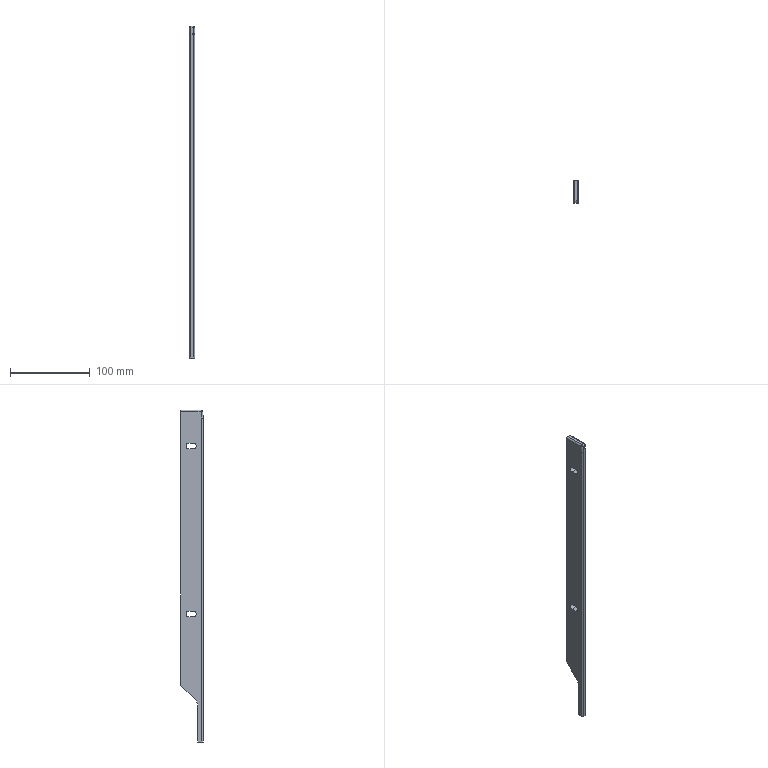Component | SolidWorks | WirePressingUnitPressingPlate-1 | 1 solid | 30 faces | box 7 x 28 x 415 mm | volume 70543 mm3 | plane 13 | cylinder 13 | sphere 4 | commonest cylinder face diameters 4 x8 7 x4 20 x1
STEP:
#1=COLOUR_RGB('',0.7922,0.8196,0.9333);
#2=FILL_AREA_STYLE_COLOUR('',#1);
#3=FILL_AREA_STYLE('',(#2));
#4=SURFACE_STYLE_FILL_AREA(#3);
#5=SURFACE_SIDE_STYLE('',(#4));
#6=SURFACE_STYLE_USAGE(.BOTH.,#5);
#7=PRESENTATION_STYLE_ASSIGNMENT((#6));
#8=CARTESIAN_POINT('',(-0.3085,-0.6154,-14.209));
#9=VERTEX_POINT('',#8);
#10=CARTESIAN_POINT('',(-0.3085,-0.8123,-14.209));
#11=VERTEX_POINT('',#10);
#12=CARTESIAN_POINT('',(-0.3085,0.2113,-14.209));
#13=DIRECTION('',(0.,-1.,-0.));
#14=VECTOR('',#13,39.37);
#15=LINE('',#12,#14);
#16=EDGE_CURVE('',#9,#11,#15,.T.);
#17=ORIENTED_EDGE('',*,*,#16,.F.);
#18=CARTESIAN_POINT('',(-0.03288,-0.6154,-14.209));
#19=VERTEX_POINT('',#18);
#20=CARTESIAN_POINT('',(-0.03288,-0.6154,-14.209));
#21=DIRECTION('',(-1.,-0.,-0.));
#22=VECTOR('',#21,39.37);
#23=LINE('',#20,#22);
#24=EDGE_CURVE('',#19,#9,#23,.T.);
#25=ORIENTED_EDGE('',*,*,#24,.F.);
#26=CARTESIAN_POINT('',(-0.03288,-0.8123,-14.209));
#27=VERTEX_POINT('',#26);
#28=CARTESIAN_POINT('',(-0.03288,0.2113,-14.209));
#29=DIRECTION('',(0.,-1.,-0.));
#30=VECTOR('',#29,39.37);
#31=LINE('',#28,#30);
#32=EDGE_CURVE('',#19,#27,#31,.T.);
#33=ORIENTED_EDGE('',*,*,#32,.T.);
#34=CARTESIAN_POINT('',(-0.1116,-0.891,-14.209));
#35=VERTEX_POINT('',#34);
#36=CARTESIAN_POINT('',(-0.1116,-0.8123,-14.209));
#37=DIRECTION('',(0.,0.,-1.));
#38=DIRECTION('',(1.,0.,0.));
#39=AXIS2_PLACEMENT_3D('',#36,#37,#38);
#40=CIRCLE('',#39,0.07874);
#41=EDGE_CURVE('',#27,#35,#40,.T.);
#42=ORIENTED_EDGE('',*,*,#41,.T.);
#43=CARTESIAN_POINT('',(-0.2297,-0.891,-14.209));
#44=VERTEX_POINT('',#43);
#45=CARTESIAN_POINT('',(-0.3085,-0.891,-14.209));
#46=DIRECTION('',(1.,0.,0.));
#47=VECTOR('',#46,39.37);
#48=LINE('',#45,#47);
#49=EDGE_CURVE('',#44,#35,#48,.T.);
#50=ORIENTED_EDGE('',*,*,#49,.F.);
#51=CARTESIAN_POINT('',(-0.2297,-0.8123,-14.209));
#52=DIRECTION('',(0.,0.,-1.));
#53=DIRECTION('',(1.,0.,0.));
#54=AXIS2_PLACEMENT_3D('',#51,#52,#53);
#55=CIRCLE('',#54,0.07874);
#56=EDGE_CURVE('',#44,#11,#55,.T.);
#57=ORIENTED_EDGE('',*,*,#56,.T.);
#58=EDGE_LOOP('',(#17,#25,#33,#42,#50,#57));
#59=FACE_OUTER_BOUND('',#58,.T.);
#60=CARTESIAN_POINT('',(-0.3085,0.2113,-14.209));
#61=DIRECTION('',(-0.,-0.,1.));
#62=DIRECTION('',(1.,0.,0.));
#63=AXIS2_PLACEMENT_3D('',#60,#61,#62);
#64=PLANE('',#63);
#65=ADVANCED_FACE('',(#59),#64,.F.);
#66=ORIENTED_EDGE('',*,*,#49,.T.);
#67=CARTESIAN_POINT('',(-0.1116,-0.891,1.732));
#68=VERTEX_POINT('',#67);
#69=CARTESIAN_POINT('',(-0.1116,-0.891,-14.209));
#70=DIRECTION('',(-0.,-0.,1.));
#71=VECTOR('',#70,39.37);
#72=LINE('',#69,#71);
#73=EDGE_CURVE('',#35,#68,#72,.T.);
#74=ORIENTED_EDGE('',*,*,#73,.T.);
#75=CARTESIAN_POINT('',(-0.2297,-0.891,1.732));
#76=VERTEX_POINT('',#75);
#77=CARTESIAN_POINT('',(-0.3085,-0.891,1.732));
#78=DIRECTION('',(-1.,-0.,-0.));
#79=VECTOR('',#78,39.37);
#80=LINE('',#77,#79);
#81=EDGE_CURVE('',#68,#76,#80,.T.);
#82=ORIENTED_EDGE('',*,*,#81,.T.);
#83=CARTESIAN_POINT('',(-0.2297,-0.891,-14.209));
#84=DIRECTION('',(0.,0.,-1.));
#85=VECTOR('',#84,39.37);
#86=LINE('',#83,#85);
#87=EDGE_CURVE('',#76,#44,#86,.T.);
#88=ORIENTED_EDGE('',*,*,#87,.T.);
#89=EDGE_LOOP('',(#66,#74,#82,#88));
#90=FACE_OUTER_BOUND('',#89,.T.);
#91=CARTESIAN_POINT('',(-0.3085,-0.891,-14.209));
#92=DIRECTION('',(-0.,1.,0.));
#93=DIRECTION('',(-1.,-0.,-0.));
#94=AXIS2_PLACEMENT_3D('',#91,#92,#93);
#95=PLANE('',#94);
#96=ADVANCED_FACE('',(#90),#95,.F.);
#97=CARTESIAN_POINT('',(-0.2297,-0.8907,1.739));
#98=VERTEX_POINT('',#97);
#99=CARTESIAN_POINT('',(-0.1116,-0.8907,1.739));
#100=VERTEX_POINT('',#99);
#101=CARTESIAN_POINT('',(-0.3085,-0.8907,1.739));
#102=DIRECTION('',(1.,0.,0.));
#103=VECTOR('',#102,39.37);
#104=LINE('',#101,#103);
#105=EDGE_CURVE('',#98,#100,#104,.T.);
#106=ORIENTED_EDGE('',*,*,#105,.T.);
#107=CARTESIAN_POINT('',(-0.1116,-0.8629,2.057));
#108=VERTEX_POINT('',#107);
#109=CARTESIAN_POINT('',(-0.1116,-0.8566,2.129));
#110=DIRECTION('',(-0.,0.08716,0.9962));
#111=VECTOR('',#110,39.37);
#112=LINE('',#109,#111);
#113=EDGE_CURVE('',#100,#108,#112,.T.);
#114=ORIENTED_EDGE('',*,*,#113,.T.);
#115=CARTESIAN_POINT('',(-0.2297,-0.8629,2.057));
#116=VERTEX_POINT('',#115);
#117=CARTESIAN_POINT('',(-0.3085,-0.8629,2.057));
#118=DIRECTION('',(-1.,-0.,-0.));
#119=VECTOR('',#118,39.37);
#120=LINE('',#117,#119);
#121=EDGE_CURVE('',#108,#116,#120,.T.);
#122=ORIENTED_EDGE('',*,*,#121,.T.);
#123=CARTESIAN_POINT('',(-0.2297,-0.8907,1.739));
#124=DIRECTION('',(0.,-0.08716,-0.9962));
#125=VECTOR('',#124,39.37);
#126=LINE('',#123,#125);
#127=EDGE_CURVE('',#116,#98,#126,.T.);
#128=ORIENTED_EDGE('',*,*,#127,.T.);
#129=EDGE_LOOP('',(#106,#114,#122,#128));
#130=FACE_OUTER_BOUND('',#129,.T.);
#131=CARTESIAN_POINT('',(-0.3085,-0.8566,2.129));
#132=DIRECTION('',(-0.,0.9962,-0.08716));
#133=DIRECTION('',(0.,-0.08716,-0.9962));
#134=AXIS2_PLACEMENT_3D('',#131,#132,#133);
#135=PLANE('',#134);
#136=ADVANCED_FACE('',(#130),#135,.F.);
#137=CARTESIAN_POINT('',(-0.2297,-0.7844,2.129));
#138=VERTEX_POINT('',#137);
#139=CARTESIAN_POINT('',(-0.1116,-0.7844,2.129));
#140=VERTEX_POINT('',#139);
#141=CARTESIAN_POINT('',(-0.3085,-0.7844,2.129));
#142=DIRECTION('',(1.,0.,0.));
#143=VECTOR('',#142,39.37);
#144=LINE('',#141,#143);
#145=EDGE_CURVE('',#138,#140,#144,.T.);
#146=ORIENTED_EDGE('',*,*,#145,.T.);
#147=CARTESIAN_POINT('',(-0.1116,0.2113,2.129));
#148=VERTEX_POINT('',#147);
#149=CARTESIAN_POINT('',(-0.1116,0.2113,2.129));
#150=DIRECTION('',(-0.,1.,0.));
#151=VECTOR('',#150,39.37);
#152=LINE('',#149,#151);
#153=EDGE_CURVE('',#140,#148,#152,.T.);
#154=ORIENTED_EDGE('',*,*,#153,.T.);
#155=CARTESIAN_POINT('',(-0.2297,0.2113,2.129));
#156=VERTEX_POINT('',#155);
#157=CARTESIAN_POINT('',(-0.3085,0.2113,2.129));
#158=DIRECTION('',(1.,0.,0.));
#159=VECTOR('',#158,39.37);
#160=LINE('',#157,#159);
#161=EDGE_CURVE('',#156,#148,#160,.T.);
#162=ORIENTED_EDGE('',*,*,#161,.F.);
#163=CARTESIAN_POINT('',(-0.2297,-0.7844,2.129));
#164=DIRECTION('',(0.,-1.,-0.));
#165=VECTOR('',#164,39.37);
#166=LINE('',#163,#165);
#167=EDGE_CURVE('',#156,#138,#166,.T.);
#168=ORIENTED_EDGE('',*,*,#167,.T.);
#169=EDGE_LOOP('',(#146,#154,#162,#168));
#170=FACE_OUTER_BOUND('',#169,.T.);
#171=CARTESIAN_POINT('',(-0.3085,0.2113,2.129));
#172=DIRECTION('',(0.,0.,-1.));
#173=DIRECTION('',(-1.,-0.,-0.));
#174=AXIS2_PLACEMENT_3D('',#171,#172,#173);
#175=PLANE('',#174);
#176=ADVANCED_FACE('',(#170),#175,.F.);
#177=CARTESIAN_POINT('',(-0.03288,0.2113,2.051));
#178=VERTEX_POINT('',#177);
#179=CARTESIAN_POINT('',(-0.03288,0.2113,-11.414));
#180=VERTEX_POINT('',#179);
#181=CARTESIAN_POINT('',(-0.03288,0.2113,-14.209));
#182=DIRECTION('',(0.,0.,-1.));
#183=VECTOR('',#182,39.37);
#184=LINE('',#181,#183);
#185=EDGE_CURVE('',#178,#180,#184,.T.);
#186=ORIENTED_EDGE('',*,*,#185,.T.);
#187=CARTESIAN_POINT('',(-0.3085,0.2113,-11.414));
#188=VERTEX_POINT('',#187);
#189=CARTESIAN_POINT('',(-0.03288,0.2113,-11.414));
#190=DIRECTION('',(-1.,-0.,-0.));
#191=VECTOR('',#190,39.37);
#192=LINE('',#189,#191);
#193=EDGE_CURVE('',#180,#188,#192,.T.);
#194=ORIENTED_EDGE('',*,*,#193,.T.);
#195=CARTESIAN_POINT('',(-0.3085,0.2113,2.051));
#196=VERTEX_POINT('',#195);
#197=CARTESIAN_POINT('',(-0.3085,0.2113,-14.209));
#198=DIRECTION('',(0.,0.,-1.));
#199=VECTOR('',#198,39.37);
#200=LINE('',#197,#199);
#201=EDGE_CURVE('',#196,#188,#200,.T.);
#202=ORIENTED_EDGE('',*,*,#201,.F.);
#203=CARTESIAN_POINT('',(-0.2297,0.2113,2.051));
#204=DIRECTION('',(-0.,1.,0.));
#205=DIRECTION('',(1.,0.,0.));
#206=AXIS2_PLACEMENT_3D('',#203,#204,#205);
#207=CIRCLE('',#206,0.07874);
#208=EDGE_CURVE('',#196,#156,#207,.T.);
#209=ORIENTED_EDGE('',*,*,#208,.T.);
#210=ORIENTED_EDGE('',*,*,#161,.T.);
#211=CARTESIAN_POINT('',(-0.1116,0.2113,2.051));
#212=DIRECTION('',(-0.,1.,0.));
#213=DIRECTION('',(1.,0.,0.));
#214=AXIS2_PLACEMENT_3D('',#211,#212,#213);
#215=CIRCLE('',#214,0.07874);
#216=EDGE_CURVE('',#148,#178,#215,.T.);
#217=ORIENTED_EDGE('',*,*,#216,.T.);
#218=EDGE_LOOP('',(#186,#194,#202,#209,#210,#217));
#219=FACE_OUTER_BOUND('',#218,.T.);
#220=CARTESIAN_POINT('',(-0.3085,0.2113,-14.209));
#221=DIRECTION('',(0.,-1.,-0.));
#222=DIRECTION('',(1.,0.,0.));
#223=AXIS2_PLACEMENT_3D('',#220,#221,#222);
#224=PLANE('',#223);
#225=ADVANCED_FACE('',(#219),#224,.F.);
#226=CARTESIAN_POINT('',(-0.3085,-0.5001,-12.125));
#227=VERTEX_POINT('',#226);
#228=CARTESIAN_POINT('',(-0.3085,0.2113,-11.414));
#229=DIRECTION('',(-0.,0.7071,0.7071));
#230=VECTOR('',#229,39.37);
#231=LINE('',#228,#230);
#232=EDGE_CURVE('',#227,#188,#231,.T.);
#233=ORIENTED_EDGE('',*,*,#232,.F.);
#234=CARTESIAN_POINT('',(-0.3085,-0.6154,-12.404));
#235=VERTEX_POINT('',#234);
#236=CARTESIAN_POINT('',(-0.3085,-0.2217,-12.404));
#237=DIRECTION('',(-1.,-0.,-0.));
#238=DIRECTION('',(0.,0.,1.));
#239=AXIS2_PLACEMENT_3D('',#236,#237,#238);
#240=CIRCLE('',#239,0.3937);
#241=EDGE_CURVE('',#235,#227,#240,.T.);
#242=ORIENTED_EDGE('',*,*,#241,.F.);
#243=CARTESIAN_POINT('',(-0.3085,-0.6154,-14.209));
#244=DIRECTION('',(-0.,-0.,1.));
#245=VECTOR('',#244,39.37);
#246=LINE('',#243,#245);
#247=EDGE_CURVE('',#9,#235,#246,.T.);
#248=ORIENTED_EDGE('',*,*,#247,.F.);
#249=ORIENTED_EDGE('',*,*,#16,.T.);
#250=CARTESIAN_POINT('',(-0.3085,-0.8123,1.732));
#251=VERTEX_POINT('',#250);
#252=CARTESIAN_POINT('',(-0.3085,-0.8123,1.732));
#253=DIRECTION('',(-0.,-0.,1.));
#254=VECTOR('',#253,39.37);
#255=LINE('',#252,#254);
#256=EDGE_CURVE('',#11,#251,#255,.T.);
#257=ORIENTED_EDGE('',*,*,#256,.T.);
#258=CARTESIAN_POINT('',(-0.3085,-0.7844,2.051));
#259=VERTEX_POINT('',#258);
#260=CARTESIAN_POINT('',(-0.3085,-0.7844,2.051));
#261=DIRECTION('',(-0.,0.08716,0.9962));
#262=VECTOR('',#261,39.37);
#263=LINE('',#260,#262);
#264=EDGE_CURVE('',#251,#259,#263,.T.);
#265=ORIENTED_EDGE('',*,*,#264,.T.);
#266=CARTESIAN_POINT('',(-0.3085,0.2113,2.051));
#267=DIRECTION('',(-0.,1.,0.));
#268=VECTOR('',#267,39.37);
#269=LINE('',#266,#268);
#270=EDGE_CURVE('',#259,#196,#269,.T.);
#271=ORIENTED_EDGE('',*,*,#270,.T.);
#272=ORIENTED_EDGE('',*,*,#201,.T.);
#273=EDGE_LOOP('',(#233,#242,#248,#249,#257,#265,#271,#272));
#274=FACE_OUTER_BOUND('',#273,.T.);
#275=CARTESIAN_POINT('',(-0.3085,-0.1824,-7.772));
#276=VERTEX_POINT('',#275);
#277=CARTESIAN_POINT('',(-0.3085,-0.1824,-8.048));
#278=VERTEX_POINT('',#277);
#279=CARTESIAN_POINT('',(-0.3085,-0.1824,-7.91));
#280=DIRECTION('',(-1.,-0.,-0.));
#281=DIRECTION('',(0.,0.,1.));
#282=AXIS2_PLACEMENT_3D('',#279,#280,#281);
#283=CIRCLE('',#282,0.1378);
#284=EDGE_CURVE('',#276,#278,#283,.T.);
#285=ORIENTED_EDGE('',*,*,#284,.F.);
#286=CARTESIAN_POINT('',(-0.3085,-0.4186,-7.772));
#287=VERTEX_POINT('',#286);
#288=CARTESIAN_POINT('',(-0.3085,-0.1824,-7.772));
#289=DIRECTION('',(-0.,1.,0.));
#290=VECTOR('',#289,39.37);
#291=LINE('',#288,#290);
#292=EDGE_CURVE('',#287,#276,#291,.T.);
#293=ORIENTED_EDGE('',*,*,#292,.F.);
#294=CARTESIAN_POINT('',(-0.3085,-0.4186,-8.048));
#295=VERTEX_POINT('',#294);
#296=CARTESIAN_POINT('',(-0.3085,-0.4186,-7.91));
#297=DIRECTION('',(-1.,-0.,-0.));
#298=DIRECTION('',(0.,0.,1.));
#299=AXIS2_PLACEMENT_3D('',#296,#297,#298);
#300=CIRCLE('',#299,0.1378);
#301=EDGE_CURVE('',#295,#287,#300,.T.);
#302=ORIENTED_EDGE('',*,*,#301,.F.);
#303=CARTESIAN_POINT('',(-0.3085,-0.1824,-8.048));
#304=DIRECTION('',(0.,-1.,-0.));
#305=VECTOR('',#304,39.37);
#306=LINE('',#303,#305);
#307=EDGE_CURVE('',#278,#295,#306,.T.);
#308=ORIENTED_EDGE('',*,*,#307,.F.);
#309=EDGE_LOOP('',(#285,#293,#302,#308));
#310=FACE_BOUND('',#309,.T.);
#311=CARTESIAN_POINT('',(-0.3085,-0.1824,0.4955));
#312=VERTEX_POINT('',#311);
#313=CARTESIAN_POINT('',(-0.3085,-0.1824,0.2199));
#314=VERTEX_POINT('',#313);
#315=CARTESIAN_POINT('',(-0.3085,-0.1824,0.3577));
#316=DIRECTION('',(-1.,-0.,-0.));
#317=DIRECTION('',(0.,0.,1.));
#318=AXIS2_PLACEMENT_3D('',#315,#316,#317);
#319=CIRCLE('',#318,0.1378);
#320=EDGE_CURVE('',#312,#314,#319,.T.);
#321=ORIENTED_EDGE('',*,*,#320,.F.);
#322=CARTESIAN_POINT('',(-0.3085,-0.4186,0.4955));
#323=VERTEX_POINT('',#322);
#324=CARTESIAN_POINT('',(-0.3085,-0.1824,0.4955));
#325=DIRECTION('',(-0.,1.,0.));
#326=VECTOR('',#325,39.37);
#327=LINE('',#324,#326);
#328=EDGE_CURVE('',#323,#312,#327,.T.);
#329=ORIENTED_EDGE('',*,*,#328,.F.);
#330=CARTESIAN_POINT('',(-0.3085,-0.4186,0.2199));
#331=VERTEX_POINT('',#330);
#332=CARTESIAN_POINT('',(-0.3085,-0.4186,0.3577));
#333=DIRECTION('',(-1.,-0.,-0.));
#334=DIRECTION('',(0.,0.,1.));
#335=AXIS2_PLACEMENT_3D('',#332,#333,#334);
#336=CIRCLE('',#335,0.1378);
#337=EDGE_CURVE('',#331,#323,#336,.T.);
#338=ORIENTED_EDGE('',*,*,#337,.F.);
#339=CARTESIAN_POINT('',(-0.3085,-0.1824,0.2199));
#340=DIRECTION('',(0.,-1.,-0.));
#341=VECTOR('',#340,39.37);
#342=LINE('',#339,#341);
#343=EDGE_CURVE('',#314,#331,#342,.T.);
#344=ORIENTED_EDGE('',*,*,#343,.F.);
#345=EDGE_LOOP('',(#321,#329,#338,#344));
#346=FACE_BOUND('',#345,.T.);
#347=CARTESIAN_POINT('',(-0.3085,-0.3398,-6.04));
#348=DIRECTION('',(-1.,-0.,-0.));
#349=DIRECTION('',(-0.,-0.,1.));
#350=AXIS2_PLACEMENT_3D('',#347,#348,#349);
#351=PLANE('',#350);
#352=ADVANCED_FACE('',(#274,#310,#346),#351,.T.);
#353=CARTESIAN_POINT('',(-0.03288,-0.4186,-7.772));
#354=VERTEX_POINT('',#353);
#355=CARTESIAN_POINT('',(-0.03288,-0.1824,-7.772));
#356=VERTEX_POINT('',#355);
#357=CARTESIAN_POINT('',(-0.03288,-0.3398,-7.772));
#358=DIRECTION('',(-0.,1.,0.));
#359=VECTOR('',#358,39.37);
#360=LINE('',#357,#359);
#361=EDGE_CURVE('',#354,#356,#360,.T.);
#362=ORIENTED_EDGE('',*,*,#361,.T.);
#363=CARTESIAN_POINT('',(-0.03288,-0.1824,-8.048));
#364=VERTEX_POINT('',#363);
#365=CARTESIAN_POINT('',(-0.03288,-0.1824,-7.91));
#366=DIRECTION('',(-1.,-0.,-0.));
#367=DIRECTION('',(0.,0.,1.));
#368=AXIS2_PLACEMENT_3D('',#365,#366,#367);
#369=CIRCLE('',#368,0.1378);
#370=EDGE_CURVE('',#356,#364,#369,.T.);
#371=ORIENTED_EDGE('',*,*,#370,.T.);
#372=CARTESIAN_POINT('',(-0.03288,-0.4186,-8.048));
#373=VERTEX_POINT('',#372);
#374=CARTESIAN_POINT('',(-0.03288,-0.3398,-8.048));
#375=DIRECTION('',(0.,-1.,-0.));
#376=VECTOR('',#375,39.37);
#377=LINE('',#374,#376);
#378=EDGE_CURVE('',#364,#373,#377,.T.);
#379=ORIENTED_EDGE('',*,*,#378,.T.);
#380=CARTESIAN_POINT('',(-0.03288,-0.4186,-7.91));
#381=DIRECTION('',(-1.,-0.,-0.));
#382=DIRECTION('',(0.,0.,1.));
#383=AXIS2_PLACEMENT_3D('',#380,#381,#382);
#384=CIRCLE('',#383,0.1378);
#385=EDGE_CURVE('',#373,#354,#384,.T.);
#386=ORIENTED_EDGE('',*,*,#385,.T.);
#387=EDGE_LOOP('',(#362,#371,#379,#386));
#388=FACE_BOUND('',#387,.T.);
#389=CARTESIAN_POINT('',(-0.03288,-0.4186,0.4955));
#390=VERTEX_POINT('',#389);
#391=CARTESIAN_POINT('',(-0.03288,-0.1824,0.4955));
#392=VERTEX_POINT('',#391);
#393=CARTESIAN_POINT('',(-0.03288,-0.3398,0.4955));
#394=DIRECTION('',(-0.,1.,0.));
#395=VECTOR('',#394,39.37);
#396=LINE('',#393,#395);
#397=EDGE_CURVE('',#390,#392,#396,.T.);
#398=ORIENTED_EDGE('',*,*,#397,.T.);
#399=CARTESIAN_POINT('',(-0.03288,-0.1824,0.2199));
#400=VERTEX_POINT('',#399);
#401=CARTESIAN_POINT('',(-0.03288,-0.1824,0.3577));
#402=DIRECTION('',(-1.,-0.,-0.));
#403=DIRECTION('',(0.,0.,1.));
#404=AXIS2_PLACEMENT_3D('',#401,#402,#403);
#405=CIRCLE('',#404,0.1378);
#406=EDGE_CURVE('',#392,#400,#405,.T.);
#407=ORIENTED_EDGE('',*,*,#406,.T.);
#408=CARTESIAN_POINT('',(-0.03288,-0.4186,0.2199));
#409=VERTEX_POINT('',#408);
#410=CARTESIAN_POINT('',(-0.03288,-0.3398,0.2199));
#411=DIRECTION('',(0.,-1.,-0.));
#412=VECTOR('',#411,39.37);
#413=LINE('',#410,#412);
#414=EDGE_CURVE('',#400,#409,#413,.T.);
#415=ORIENTED_EDGE('',*,*,#414,.T.);
#416=CARTESIAN_POINT('',(-0.03288,-0.4186,0.3577));
#417=DIRECTION('',(-1.,-0.,-0.));
#418=DIRECTION('',(0.,0.,1.));
#419=AXIS2_PLACEMENT_3D('',#416,#417,#418);
#420=CIRCLE('',#419,0.1378);
#421=EDGE_CURVE('',#409,#390,#420,.T.);
#422=ORIENTED_EDGE('',*,*,#421,.T.);
#423=EDGE_LOOP('',(#398,#407,#415,#422));
#424=FACE_BOUND('',#423,.T.);
#425=CARTESIAN_POINT('',(-0.03288,-0.6154,-12.404));
#426=VERTEX_POINT('',#425);
#427=CARTESIAN_POINT('',(-0.03288,-0.5001,-12.125));
#428=VERTEX_POINT('',#427);
#429=CARTESIAN_POINT('',(-0.03288,-0.2217,-12.404));
#430=DIRECTION('',(-1.,-0.,-0.));
#431=DIRECTION('',(-0.,0.,1.));
#432=AXIS2_PLACEMENT_3D('',#429,#430,#431);
#433=CIRCLE('',#432,0.3937);
#434=EDGE_CURVE('',#426,#428,#433,.T.);
#435=ORIENTED_EDGE('',*,*,#434,.T.);
#436=CARTESIAN_POINT('',(-0.03288,0.2113,-11.414));
#437=DIRECTION('',(-0.,0.7071,0.7071));
#438=VECTOR('',#437,39.37);
#439=LINE('',#436,#438);
#440=EDGE_CURVE('',#428,#180,#439,.T.);
#441=ORIENTED_EDGE('',*,*,#440,.T.);
#442=ORIENTED_EDGE('',*,*,#185,.F.);
#443=CARTESIAN_POINT('',(-0.03288,-0.7844,2.051));
#444=VERTEX_POINT('',#443);
#445=CARTESIAN_POINT('',(-0.03288,-0.3398,2.051));
#446=DIRECTION('',(0.,-1.,-0.));
#447=VECTOR('',#446,39.37);
#448=LINE('',#445,#447);
#449=EDGE_CURVE('',#178,#444,#448,.T.);
#450=ORIENTED_EDGE('',*,*,#449,.T.);
#451=CARTESIAN_POINT('',(-0.03288,-0.8123,1.732));
#452=VERTEX_POINT('',#451);
#453=CARTESIAN_POINT('',(-0.03288,-1.483,-5.94));
#454=DIRECTION('',(0.,-0.08716,-0.9962));
#455=VECTOR('',#454,39.37);
#456=LINE('',#453,#455);
#457=EDGE_CURVE('',#444,#452,#456,.T.);
#458=ORIENTED_EDGE('',*,*,#457,.T.);
#459=CARTESIAN_POINT('',(-0.03288,-0.8123,-6.04));
#460=DIRECTION('',(0.,0.,-1.));
#461=VECTOR('',#460,39.37);
#462=LINE('',#459,#461);
#463=EDGE_CURVE('',#452,#27,#462,.T.);
#464=ORIENTED_EDGE('',*,*,#463,.T.);
#465=ORIENTED_EDGE('',*,*,#32,.F.);
#466=CARTESIAN_POINT('',(-0.03288,-0.6154,-14.209));
#467=DIRECTION('',(-0.,-0.,1.));
#468=VECTOR('',#467,39.37);
#469=LINE('',#466,#468);
#470=EDGE_CURVE('',#19,#426,#469,.T.);
#471=ORIENTED_EDGE('',*,*,#470,.T.);
#472=EDGE_LOOP('',(#435,#441,#442,#450,#458,#464,#465,#471));
#473=FACE_OUTER_BOUND('',#472,.T.);
#474=CARTESIAN_POINT('',(-0.03288,-0.3398,-6.04));
#475=DIRECTION('',(-1.,-0.,-0.));
#476=DIRECTION('',(-0.,-0.,1.));
#477=AXIS2_PLACEMENT_3D('',#474,#475,#476);
#478=PLANE('',#477);
#479=ADVANCED_FACE('',(#388,#424,#473),#478,.F.);
#480=ORIENTED_EDGE('',*,*,#81,.F.);
#481=CARTESIAN_POINT('',(-0.1116,-0.8123,1.732));
#482=DIRECTION('',(-1.,-0.,-0.));
#483=DIRECTION('',(0.,0.,-1.));
#484=AXIS2_PLACEMENT_3D('',#481,#482,#483);
#485=CIRCLE('',#484,0.07874);
#486=EDGE_CURVE('',#68,#100,#485,.T.);
#487=ORIENTED_EDGE('',*,*,#486,.T.);
#488=ORIENTED_EDGE('',*,*,#105,.F.);
#489=CARTESIAN_POINT('',(-0.2297,-0.8123,1.732));
#490=DIRECTION('',(1.,0.,0.));
#491=DIRECTION('',(0.,0.,-1.));
#492=AXIS2_PLACEMENT_3D('',#489,#490,#491);
#493=CIRCLE('',#492,0.07874);
#494=EDGE_CURVE('',#98,#76,#493,.T.);
#495=ORIENTED_EDGE('',*,*,#494,.T.);
#496=EDGE_LOOP('',(#480,#487,#488,#495));
#497=FACE_OUTER_BOUND('',#496,.T.);
#498=CARTESIAN_POINT('',(-0.3085,-0.8123,1.732));
#499=DIRECTION('',(1.,0.,0.));
#500=DIRECTION('',(0.,0.,-1.));
#501=AXIS2_PLACEMENT_3D('',#498,#499,#500);
#502=CYLINDRICAL_SURFACE('',#501,0.07874);
#503=ADVANCED_FACE('',(#497),#502,.T.);
#504=ORIENTED_EDGE('',*,*,#121,.F.);
#505=CARTESIAN_POINT('',(-0.1116,-0.7844,2.051));
#506=DIRECTION('',(-1.,-0.,-0.));
#507=DIRECTION('',(0.,0.,-1.));
#508=AXIS2_PLACEMENT_3D('',#505,#506,#507);
#509=CIRCLE('',#508,0.07874);
#510=EDGE_CURVE('',#108,#140,#509,.T.);
#511=ORIENTED_EDGE('',*,*,#510,.T.);
#512=ORIENTED_EDGE('',*,*,#145,.F.);
#513=CARTESIAN_POINT('',(-0.2297,-0.7844,2.051));
#514=DIRECTION('',(1.,0.,0.));
#515=DIRECTION('',(0.,0.,-1.));
#516=AXIS2_PLACEMENT_3D('',#513,#514,#515);
#517=CIRCLE('',#516,0.07874);
#518=EDGE_CURVE('',#138,#116,#517,.T.);
#519=ORIENTED_EDGE('',*,*,#518,.T.);
#520=EDGE_LOOP('',(#504,#511,#512,#519));
#521=FACE_OUTER_BOUND('',#520,.T.);
#522=CARTESIAN_POINT('',(-0.3085,-0.7844,2.051));
#523=DIRECTION('',(1.,0.,0.));
#524=DIRECTION('',(0.,0.,-1.));
#525=AXIS2_PLACEMENT_3D('',#522,#523,#524);
#526=CYLINDRICAL_SURFACE('',#525,0.07874);
#527=ADVANCED_FACE('',(#521),#526,.T.);
#528=CARTESIAN_POINT('',(-0.1116,-0.8123,1.732));
#529=DIRECTION('',(-0.,-0.,1.));
#530=DIRECTION('',(1.,0.,0.));
#531=AXIS2_PLACEMENT_3D('',#528,#529,#530);
#532=CIRCLE('',#531,0.07874);
#533=EDGE_CURVE('',#68,#452,#532,.T.);
#534=ORIENTED_EDGE('',*,*,#533,.F.);
#535=ORIENTED_EDGE('',*,*,#73,.F.);
#536=ORIENTED_EDGE('',*,*,#41,.F.);
#537=ORIENTED_EDGE('',*,*,#463,.F.);
#538=EDGE_LOOP('',(#534,#535,#536,#537));
#539=FACE_OUTER_BOUND('',#538,.T.);
#540=CARTESIAN_POINT('',(-0.1116,-0.8123,-14.209));
#541=DIRECTION('',(-0.,-0.,1.));
#542=DIRECTION('',(1.,0.,0.));
#543=AXIS2_PLACEMENT_3D('',#540,#541,#542);
#544=CYLINDRICAL_SURFACE('',#543,0.07874);
#545=ADVANCED_FACE('',(#539),#544,.T.);
#546=ORIENTED_EDGE('',*,*,#486,.F.);
#547=ORIENTED_EDGE('',*,*,#533,.T.);
#548=CARTESIAN_POINT('',(-0.1116,-0.8123,1.732));
#549=DIRECTION('',(-0.,0.08716,0.9962));
#550=DIRECTION('',(0.,0.9962,-0.08716));
#551=AXIS2_PLACEMENT_3D('',#548,#549,#550);
#552=CIRCLE('',#551,0.07874);
#553=EDGE_CURVE('',#100,#452,#552,.T.);
#554=ORIENTED_EDGE('',*,*,#553,.F.);
#555=EDGE_LOOP('',(#546,#547,#554));
#556=FACE_OUTER_BOUND('',#555,.T.);
#557=CARTESIAN_POINT('',(-0.1116,-0.8123,1.732));
#558=DIRECTION('',(-0.,1.,0.));
#559=DIRECTION('',(0.,0.,1.));
#560=AXIS2_PLACEMENT_3D('',#557,#558,#559);
#561=SPHERICAL_SURFACE('',#560,0.07874);
#562=ADVANCED_FACE('',(#556),#561,.T.);
#563=CARTESIAN_POINT('',(-0.1116,-0.7844,2.051));
#564=DIRECTION('',(0.,0.08716,0.9962));
#565=DIRECTION('',(0.,0.9962,-0.08716));
#566=AXIS2_PLACEMENT_3D('',#563,#564,#565);
#567=CIRCLE('',#566,0.07874);
#568=EDGE_CURVE('',#108,#444,#567,.T.);
#569=ORIENTED_EDGE('',*,*,#568,.F.);
#570=ORIENTED_EDGE('',*,*,#113,.F.);
#571=ORIENTED_EDGE('',*,*,#553,.T.);
#572=ORIENTED_EDGE('',*,*,#457,.F.);
#573=EDGE_LOOP('',(#569,#570,#571,#572));
#574=FACE_OUTER_BOUND('',#573,.T.);
#575=CARTESIAN_POINT('',(-0.1116,-0.7781,2.122));
#576=DIRECTION('',(-0.,0.08716,0.9962));
#577=DIRECTION('',(0.,0.9962,-0.08716));
#578=AXIS2_PLACEMENT_3D('',#575,#576,#577);
#579=CYLINDRICAL_SURFACE('',#578,0.07874);
#580=ADVANCED_FACE('',(#574),#579,.T.);
#581=ORIENTED_EDGE('',*,*,#510,.F.);
#582=ORIENTED_EDGE('',*,*,#568,.T.);
#583=CARTESIAN_POINT('',(-0.1116,-0.7844,2.051));
#584=DIRECTION('',(-0.,1.,0.));
#585=DIRECTION('',(-1.,0.,0.));
#586=AXIS2_PLACEMENT_3D('',#583,#584,#585);
#587=CIRCLE('',#586,0.07874);
#588=EDGE_CURVE('',#140,#444,#587,.T.);
#589=ORIENTED_EDGE('',*,*,#588,.F.);
#590=EDGE_LOOP('',(#581,#582,#589));
#591=FACE_OUTER_BOUND('',#590,.T.);
#592=CARTESIAN_POINT('',(-0.1116,-0.7844,2.051));
#593=DIRECTION('',(-0.,1.,0.));
#594=DIRECTION('',(0.,0.,1.));
#595=AXIS2_PLACEMENT_3D('',#592,#593,#594);
#596=SPHERICAL_SURFACE('',#595,0.07874);
#597=ADVANCED_FACE('',(#591),#596,.T.);
#598=ORIENTED_EDGE('',*,*,#588,.T.);
#599=ORIENTED_EDGE('',*,*,#449,.F.);
#600=ORIENTED_EDGE('',*,*,#216,.F.);
#601=ORIENTED_EDGE('',*,*,#153,.F.);
#602=EDGE_LOOP('',(#598,#599,#600,#601));
#603=FACE_OUTER_BOUND('',#602,.T.);
#604=CARTESIAN_POINT('',(-0.1116,0.2113,2.051));
#605=DIRECTION('',(-0.,1.,0.));
#606=DIRECTION('',(-1.,0.,0.));
#607=AXIS2_PLACEMENT_3D('',#604,#605,#606);
#608=CYLINDRICAL_SURFACE('',#607,0.07874);
#609=ADVANCED_FACE('',(#603),#608,.T.);
#610=ORIENTED_EDGE('',*,*,#56,.F.);
#611=ORIENTED_EDGE('',*,*,#87,.F.);
#612=CARTESIAN_POINT('',(-0.2297,-0.8123,1.732));
#613=DIRECTION('',(-0.,-0.,1.));
#614=DIRECTION('',(1.,0.,0.));
#615=AXIS2_PLACEMENT_3D('',#612,#613,#614);
#616=CIRCLE('',#615,0.07874);
#617=EDGE_CURVE('',#251,#76,#616,.T.);
#618=ORIENTED_EDGE('',*,*,#617,.F.);
#619=ORIENTED_EDGE('',*,*,#256,.F.);
#620=EDGE_LOOP('',(#610,#611,#618,#619));
#621=FACE_OUTER_BOUND('',#620,.T.);
#622=CARTESIAN_POINT('',(-0.2297,-0.8123,-6.04));
#623=DIRECTION('',(0.,0.,-1.));
#624=DIRECTION('',(-1.,0.,0.));
#625=AXIS2_PLACEMENT_3D('',#622,#623,#624);
#626=CYLINDRICAL_SURFACE('',#625,0.07874);
#627=ADVANCED_FACE('',(#621),#626,.T.);
#628=ORIENTED_EDGE('',*,*,#617,.T.);
#629=ORIENTED_EDGE('',*,*,#494,.F.);
#630=CARTESIAN_POINT('',(-0.2297,-0.8123,1.732));
#631=DIRECTION('',(-0.,0.08716,0.9962));
#632=DIRECTION('',(0.,0.9962,-0.08716));
#633=AXIS2_PLACEMENT_3D('',#630,#631,#632);
#634=CIRCLE('',#633,0.07874);
#635=EDGE_CURVE('',#251,#98,#634,.T.);
#636=ORIENTED_EDGE('',*,*,#635,.F.);
#637=EDGE_LOOP('',(#628,#629,#636));
#638=FACE_OUTER_BOUND('',#637,.T.);
#639=CARTESIAN_POINT('',(-0.2297,-0.8123,1.732));
#640=DIRECTION('',(-0.,1.,0.));
#641=DIRECTION('',(0.,0.,1.));
#642=AXIS2_PLACEMENT_3D('',#639,#640,#641);
#643=SPHERICAL_SURFACE('',#642,0.07874);
#644=ADVANCED_FACE('',(#638),#643,.T.);
#645=ORIENTED_EDGE('',*,*,#635,.T.);
#646=ORIENTED_EDGE('',*,*,#127,.F.);
#647=CARTESIAN_POINT('',(-0.2297,-0.7844,2.051));
#648=DIRECTION('',(-0.,0.08716,0.9962));
#649=DIRECTION('',(0.,0.9962,-0.08716));
#650=AXIS2_PLACEMENT_3D('',#647,#648,#649);
#651=CIRCLE('',#650,0.07874);
#652=EDGE_CURVE('',#259,#116,#651,.T.);
#653=ORIENTED_EDGE('',*,*,#652,.F.);
#654=ORIENTED_EDGE('',*,*,#264,.F.);
#655=EDGE_LOOP('',(#645,#646,#653,#654));
#656=FACE_OUTER_BOUND('',#655,.T.);
#657=CARTESIAN_POINT('',(-0.2297,-1.483,-5.94));
#658=DIRECTION('',(0.,-0.08716,-0.9962));
#659=DIRECTION('',(0.,-0.9962,0.08716));
#660=AXIS2_PLACEMENT_3D('',#657,#658,#659);
#661=CYLINDRICAL_SURFACE('',#660,0.07874);
#662=ADVANCED_FACE('',(#656),#661,.T.);
#663=ORIENTED_EDGE('',*,*,#652,.T.);
#664=ORIENTED_EDGE('',*,*,#518,.F.);
#665=CARTESIAN_POINT('',(-0.2297,-0.7844,2.051));
#666=DIRECTION('',(-0.,1.,0.));
#667=DIRECTION('',(-1.,0.,0.));
#668=AXIS2_PLACEMENT_3D('',#665,#666,#667);
#669=CIRCLE('',#668,0.07874);
#670=EDGE_CURVE('',#259,#138,#669,.T.);
#671=ORIENTED_EDGE('',*,*,#670,.F.);
#672=EDGE_LOOP('',(#663,#664,#671));
#673=FACE_OUTER_BOUND('',#672,.T.);
#674=CARTESIAN_POINT('',(-0.2297,-0.7844,2.051));
#675=DIRECTION('',(-0.,1.,0.));
#676=DIRECTION('',(0.,0.,1.));
#677=AXIS2_PLACEMENT_3D('',#674,#675,#676);
#678=SPHERICAL_SURFACE('',#677,0.07874);
#679=ADVANCED_FACE('',(#673),#678,.T.);
#680=ORIENTED_EDGE('',*,*,#670,.T.);
#681=ORIENTED_EDGE('',*,*,#167,.F.);
#682=ORIENTED_EDGE('',*,*,#208,.F.);
#683=ORIENTED_EDGE('',*,*,#270,.F.);
#684=EDGE_LOOP('',(#680,#681,#682,#683));
#685=FACE_OUTER_BOUND('',#684,.T.);
#686=CARTESIAN_POINT('',(-0.2297,-0.3398,2.051));
#687=DIRECTION('',(0.,-1.,-0.));
#688=DIRECTION('',(1.,0.,0.));
#689=AXIS2_PLACEMENT_3D('',#686,#687,#688);
#690=CYLINDRICAL_SURFACE('',#689,0.07874);
#691=ADVANCED_FACE('',(#685),#690,.T.);
#692=CARTESIAN_POINT('',(0.08523,-0.1824,0.4955));
#693=DIRECTION('',(-1.,-0.,-0.));
#694=VECTOR('',#693,39.37);
#695=LINE('',#692,#694);
#696=EDGE_CURVE('',#392,#312,#695,.T.);
#697=ORIENTED_EDGE('',*,*,#696,.T.);
#698=ORIENTED_EDGE('',*,*,#320,.T.);
#699=CARTESIAN_POINT('',(0.08523,-0.1824,0.2199));
#700=DIRECTION('',(-1.,-0.,-0.));
#701=VECTOR('',#700,39.37);
#702=LINE('',#699,#701);
#703=EDGE_CURVE('',#400,#314,#702,.T.);
#704=ORIENTED_EDGE('',*,*,#703,.F.);
#705=ORIENTED_EDGE('',*,*,#406,.F.);
#706=EDGE_LOOP('',(#697,#698,#704,#705));
#707=FACE_OUTER_BOUND('',#706,.T.);
#708=CARTESIAN_POINT('',(0.08523,-0.1824,0.3577));
#709=DIRECTION('',(-1.,-0.,-0.));
#710=DIRECTION('',(0.,0.,1.));
#711=AXIS2_PLACEMENT_3D('',#708,#709,#710);
#712=CYLINDRICAL_SURFACE('',#711,0.1378);
#713=ADVANCED_FACE('',(#707),#712,.F.);
#714=CARTESIAN_POINT('',(0.08523,-0.4186,0.4955));
#715=DIRECTION('',(-1.,-0.,-0.));
#716=VECTOR('',#715,39.37);
#717=LINE('',#714,#716);
#718=EDGE_CURVE('',#390,#323,#717,.T.);
#719=ORIENTED_EDGE('',*,*,#718,.T.);
#720=ORIENTED_EDGE('',*,*,#328,.T.);
#721=ORIENTED_EDGE('',*,*,#696,.F.);
#722=ORIENTED_EDGE('',*,*,#397,.F.);
#723=EDGE_LOOP('',(#719,#720,#721,#722));
#724=FACE_OUTER_BOUND('',#723,.T.);
#725=CARTESIAN_POINT('',(0.08523,-0.1824,0.4955));
#726=DIRECTION('',(-0.,-0.,1.));
#727=DIRECTION('',(1.,0.,0.));
#728=AXIS2_PLACEMENT_3D('',#725,#726,#727);
#729=PLANE('',#728);
#730=ADVANCED_FACE('',(#724),#729,.F.);
#731=CARTESIAN_POINT('',(0.08523,-0.4186,0.2199));
#732=DIRECTION('',(-1.,-0.,-0.));
#733=VECTOR('',#732,39.37);
#734=LINE('',#731,#733);
#735=EDGE_CURVE('',#409,#331,#734,.T.);
#736=ORIENTED_EDGE('',*,*,#735,.T.);
#737=ORIENTED_EDGE('',*,*,#337,.T.);
#738=ORIENTED_EDGE('',*,*,#718,.F.);
#739=ORIENTED_EDGE('',*,*,#421,.F.);
#740=EDGE_LOOP('',(#736,#737,#738,#739));
#741=FACE_OUTER_BOUND('',#740,.T.);
#742=CARTESIAN_POINT('',(0.08523,-0.4186,0.3577));
#743=DIRECTION('',(-1.,-0.,-0.));
#744=DIRECTION('',(0.,0.,1.));
#745=AXIS2_PLACEMENT_3D('',#742,#743,#744);
#746=CYLINDRICAL_SURFACE('',#745,0.1378);
#747=ADVANCED_FACE('',(#741),#746,.F.);
#748=ORIENTED_EDGE('',*,*,#703,.T.);
#749=ORIENTED_EDGE('',*,*,#343,.T.);
#750=ORIENTED_EDGE('',*,*,#735,.F.);
#751=ORIENTED_EDGE('',*,*,#414,.F.);
#752=EDGE_LOOP('',(#748,#749,#750,#751));
#753=FACE_OUTER_BOUND('',#752,.T.);
#754=CARTESIAN_POINT('',(0.08523,-0.1824,0.2199));
#755=DIRECTION('',(0.,0.,-1.));
#756=DIRECTION('',(-1.,-0.,-0.));
#757=AXIS2_PLACEMENT_3D('',#754,#755,#756);
#758=PLANE('',#757);
#759=ADVANCED_FACE('',(#753),#758,.F.);
#760=CARTESIAN_POINT('',(0.08523,-0.1824,-7.772));
#761=DIRECTION('',(-1.,-0.,-0.));
#762=VECTOR('',#761,39.37);
#763=LINE('',#760,#762);
#764=EDGE_CURVE('',#356,#276,#763,.T.);
#765=ORIENTED_EDGE('',*,*,#764,.T.);
#766=ORIENTED_EDGE('',*,*,#284,.T.);
#767=CARTESIAN_POINT('',(0.08523,-0.1824,-8.048));
#768=DIRECTION('',(-1.,-0.,-0.));
#769=VECTOR('',#768,39.37);
#770=LINE('',#767,#769);
#771=EDGE_CURVE('',#364,#278,#770,.T.);
#772=ORIENTED_EDGE('',*,*,#771,.F.);
#773=ORIENTED_EDGE('',*,*,#370,.F.);
#774=EDGE_LOOP('',(#765,#766,#772,#773));
#775=FACE_OUTER_BOUND('',#774,.T.);
#776=CARTESIAN_POINT('',(0.08523,-0.1824,-7.91));
#777=DIRECTION('',(-1.,-0.,-0.));
#778=DIRECTION('',(0.,0.,1.));
#779=AXIS2_PLACEMENT_3D('',#776,#777,#778);
#780=CYLINDRICAL_SURFACE('',#779,0.1378);
#781=ADVANCED_FACE('',(#775),#780,.F.);
#782=CARTESIAN_POINT('',(0.08523,-0.4186,-7.772));
#783=DIRECTION('',(-1.,-0.,-0.));
#784=VECTOR('',#783,39.37);
#785=LINE('',#782,#784);
#786=EDGE_CURVE('',#354,#287,#785,.T.);
#787=ORIENTED_EDGE('',*,*,#786,.T.);
#788=ORIENTED_EDGE('',*,*,#292,.T.);
#789=ORIENTED_EDGE('',*,*,#764,.F.);
#790=ORIENTED_EDGE('',*,*,#361,.F.);
#791=EDGE_LOOP('',(#787,#788,#789,#790));
#792=FACE_OUTER_BOUND('',#791,.T.);
#793=CARTESIAN_POINT('',(0.08523,-0.1824,-7.772));
#794=DIRECTION('',(-0.,-0.,1.));
#795=DIRECTION('',(1.,0.,0.));
#796=AXIS2_PLACEMENT_3D('',#793,#794,#795);
#797=PLANE('',#796);
#798=ADVANCED_FACE('',(#792),#797,.F.);
#799=CARTESIAN_POINT('',(0.08523,-0.4186,-8.048));
#800=DIRECTION('',(-1.,-0.,-0.));
#801=VECTOR('',#800,39.37);
#802=LINE('',#799,#801);
#803=EDGE_CURVE('',#373,#295,#802,.T.);
#804=ORIENTED_EDGE('',*,*,#803,.T.);
#805=ORIENTED_EDGE('',*,*,#301,.T.);
#806=ORIENTED_EDGE('',*,*,#786,.F.);
#807=ORIENTED_EDGE('',*,*,#385,.F.);
#808=EDGE_LOOP('',(#804,#805,#806,#807));
#809=FACE_OUTER_BOUND('',#808,.T.);
#810=CARTESIAN_POINT('',(0.08523,-0.4186,-7.91));
#811=DIRECTION('',(-1.,-0.,-0.));
#812=DIRECTION('',(0.,0.,1.));
#813=AXIS2_PLACEMENT_3D('',#810,#811,#812);
#814=CYLINDRICAL_SURFACE('',#813,0.1378);
#815=ADVANCED_FACE('',(#809),#814,.F.);
#816=ORIENTED_EDGE('',*,*,#771,.T.);
#817=ORIENTED_EDGE('',*,*,#307,.T.);
#818=ORIENTED_EDGE('',*,*,#803,.F.);
#819=ORIENTED_EDGE('',*,*,#378,.F.);
#820=EDGE_LOOP('',(#816,#817,#818,#819));
#821=FACE_OUTER_BOUND('',#820,.T.);
#822=CARTESIAN_POINT('',(0.08523,-0.1824,-8.048));
#823=DIRECTION('',(0.,0.,-1.));
#824=DIRECTION('',(-1.,-0.,-0.));
#825=AXIS2_PLACEMENT_3D('',#822,#823,#824);
#826=PLANE('',#825);
#827=ADVANCED_FACE('',(#821),#826,.F.);
#828=ORIENTED_EDGE('',*,*,#232,.T.);
#829=ORIENTED_EDGE('',*,*,#193,.F.);
#830=ORIENTED_EDGE('',*,*,#440,.F.);
#831=CARTESIAN_POINT('',(-0.03288,-0.5001,-12.125));
#832=DIRECTION('',(-1.,-0.,-0.));
#833=VECTOR('',#832,39.37);
#834=LINE('',#831,#833);
#835=EDGE_CURVE('',#428,#227,#834,.T.);
#836=ORIENTED_EDGE('',*,*,#835,.T.);
#837=EDGE_LOOP('',(#828,#829,#830,#836));
#838=FACE_OUTER_BOUND('',#837,.T.);
#839=CARTESIAN_POINT('',(-0.03288,0.2113,-11.414));
#840=DIRECTION('',(-0.,-0.7071,0.7071));
#841=DIRECTION('',(-0.,0.7071,0.7071));
#842=AXIS2_PLACEMENT_3D('',#839,#840,#841);
#843=PLANE('',#842);
#844=ADVANCED_FACE('',(#838),#843,.F.);
#845=ORIENTED_EDGE('',*,*,#241,.T.);
#846=ORIENTED_EDGE('',*,*,#835,.F.);
#847=ORIENTED_EDGE('',*,*,#434,.F.);
#848=CARTESIAN_POINT('',(-0.03288,-0.6154,-12.404));
#849=DIRECTION('',(-1.,-0.,-0.));
#850=VECTOR('',#849,39.37);
#851=LINE('',#848,#850);
#852=EDGE_CURVE('',#426,#235,#851,.T.);
#853=ORIENTED_EDGE('',*,*,#852,.T.);
#854=EDGE_LOOP('',(#845,#846,#847,#853));
#855=FACE_OUTER_BOUND('',#854,.T.);
#856=CARTESIAN_POINT('',(-0.03288,-0.2217,-12.404));
#857=DIRECTION('',(-1.,-0.,-0.));
#858=DIRECTION('',(-0.,0.,1.));
#859=AXIS2_PLACEMENT_3D('',#856,#857,#858);
#860=CYLINDRICAL_SURFACE('',#859,0.3937);
#861=ADVANCED_FACE('',(#855),#860,.F.);
#862=ORIENTED_EDGE('',*,*,#247,.T.);
#863=ORIENTED_EDGE('',*,*,#852,.F.);
#864=ORIENTED_EDGE('',*,*,#470,.F.);
#865=ORIENTED_EDGE('',*,*,#24,.T.);
#866=EDGE_LOOP('',(#862,#863,#864,#865));
#867=FACE_OUTER_BOUND('',#866,.T.);
#868=CARTESIAN_POINT('',(-0.03288,-0.6154,-14.209));
#869=DIRECTION('',(0.,-1.,-0.));
#870=DIRECTION('',(-0.,-0.,1.));
#871=AXIS2_PLACEMENT_3D('',#868,#869,#870);
#872=PLANE('',#871);
#873=ADVANCED_FACE('',(#867),#872,.F.);
#874=CLOSED_SHELL('',(#65,#96,#136,#176,#225,#352,#479,#503,#527,#545,#562,#580,#597,#609,#627,#644,#662,#679,#691,#713,#730,#747,#759,#781,#798,#815,#827,#844,#861,#873));
#875=MANIFOLD_SOLID_BREP('',#874);
#876=STYLED_ITEM('',(#7),#875);
#877=PRESENTATION_LAYER_ASSIGNMENT('','',(#876));
#878=CARTESIAN_POINT('',(0.,0.,0.));
#879=DIRECTION('',(0.,0.,1.));
#880=DIRECTION('',(1.,0.,0.));
#881=AXIS2_PLACEMENT_3D('',#878,#879,#880);
#882=(LENGTH_UNIT()NAMED_UNIT(*)SI_UNIT($,.METRE.));
#883=LENGTH_MEASURE_WITH_UNIT(LENGTH_MEASURE(0.0254),#882);
#884=DIMENSIONAL_EXPONENTS(1.,0.,0.,0.,0.,0.,0.);
#885=(CONVERSION_BASED_UNIT('',#883)LENGTH_UNIT()NAMED_UNIT(#884));
#886=UNCERTAINTY_MEASURE_WITH_UNIT(LENGTH_MEASURE(0.00001),#885,'','');
#887=(NAMED_UNIT(*)PLANE_ANGLE_UNIT()SI_UNIT($,.RADIAN.));
#888=(NAMED_UNIT(*)SI_UNIT($,.STERADIAN.)SOLID_ANGLE_UNIT());
#889=(GEOMETRIC_REPRESENTATION_CONTEXT(3)GLOBAL_UNCERTAINTY_ASSIGNED_CONTEXT((#886))GLOBAL_UNIT_ASSIGNED_CONTEXT((#885,#887,#888))REPRESENTATION_CONTEXT('',''));
#890=ADVANCED_BREP_SHAPE_REPRESENTATION('',(#875,#881),#889);
#891=(LENGTH_UNIT()NAMED_UNIT(*)SI_UNIT($,.METRE.));
#892=LENGTH_MEASURE_WITH_UNIT(LENGTH_MEASURE(0.0254),#891);
#893=DIMENSIONAL_EXPONENTS(1.,0.,0.,0.,0.,0.,0.);
#894=(CONVERSION_BASED_UNIT('',#892)LENGTH_UNIT()NAMED_UNIT(#893));
#895=UNCERTAINTY_MEASURE_WITH_UNIT(LENGTH_MEASURE(0.00001),#894,'','');
#896=(NAMED_UNIT(*)PLANE_ANGLE_UNIT()SI_UNIT($,.RADIAN.));
#897=(NAMED_UNIT(*)SI_UNIT($,.STERADIAN.)SOLID_ANGLE_UNIT());
#898=(GEOMETRIC_REPRESENTATION_CONTEXT(3)GLOBAL_UNCERTAINTY_ASSIGNED_CONTEXT((#895))GLOBAL_UNIT_ASSIGNED_CONTEXT((#894,#896,#897))REPRESENTATION_CONTEXT('',''));
#899=MECHANICAL_DESIGN_GEOMETRIC_PRESENTATION_REPRESENTATION('',(#876),#898);